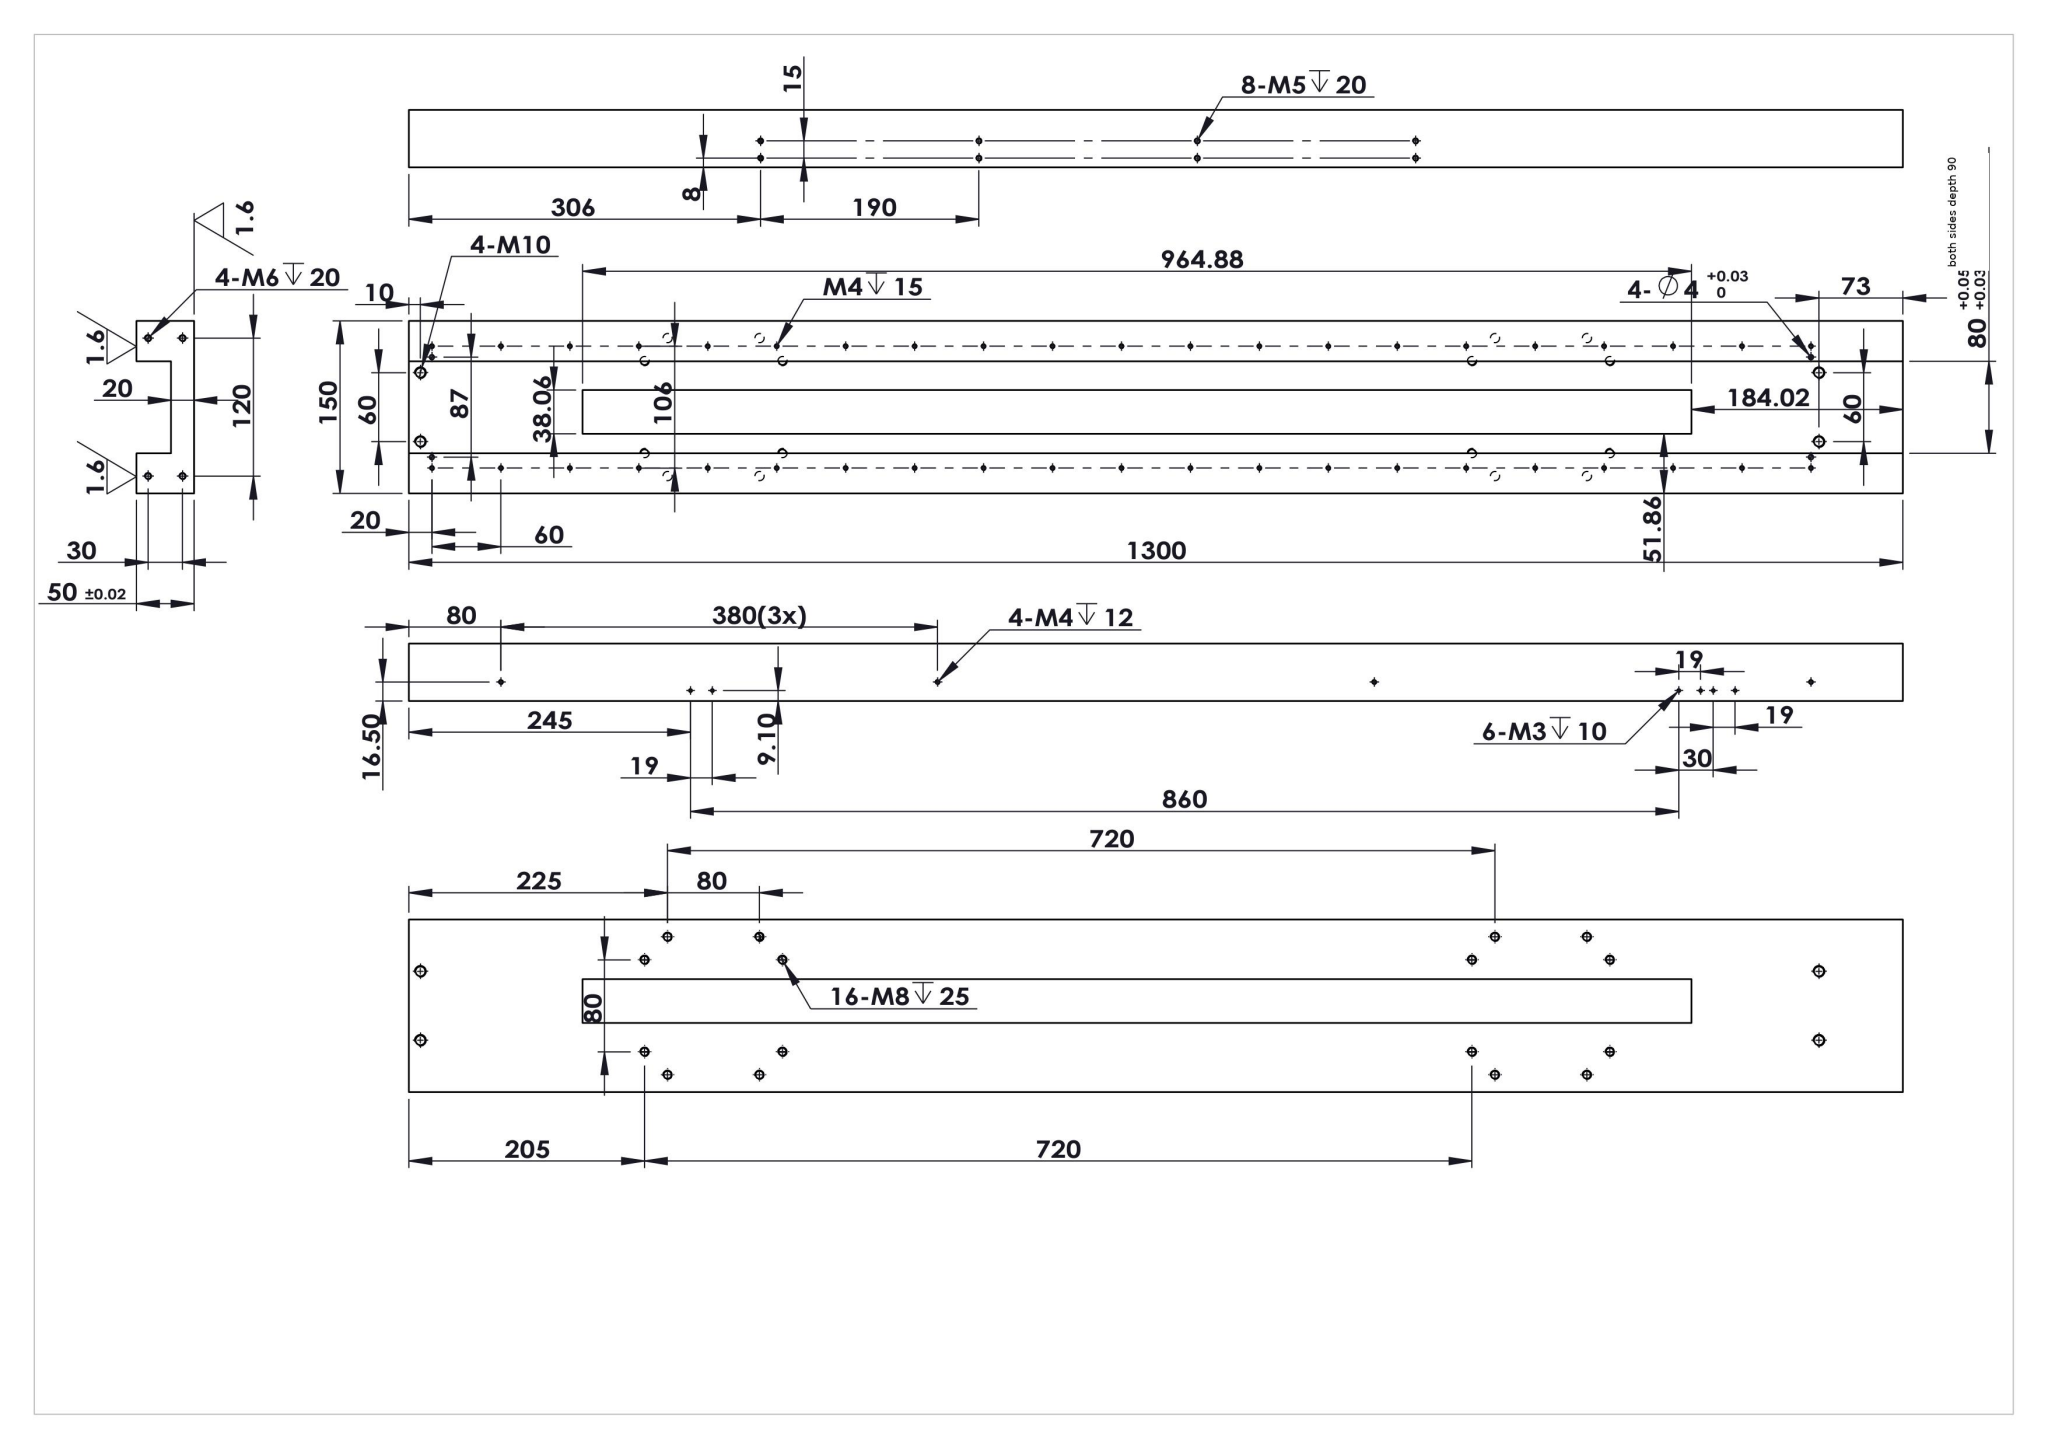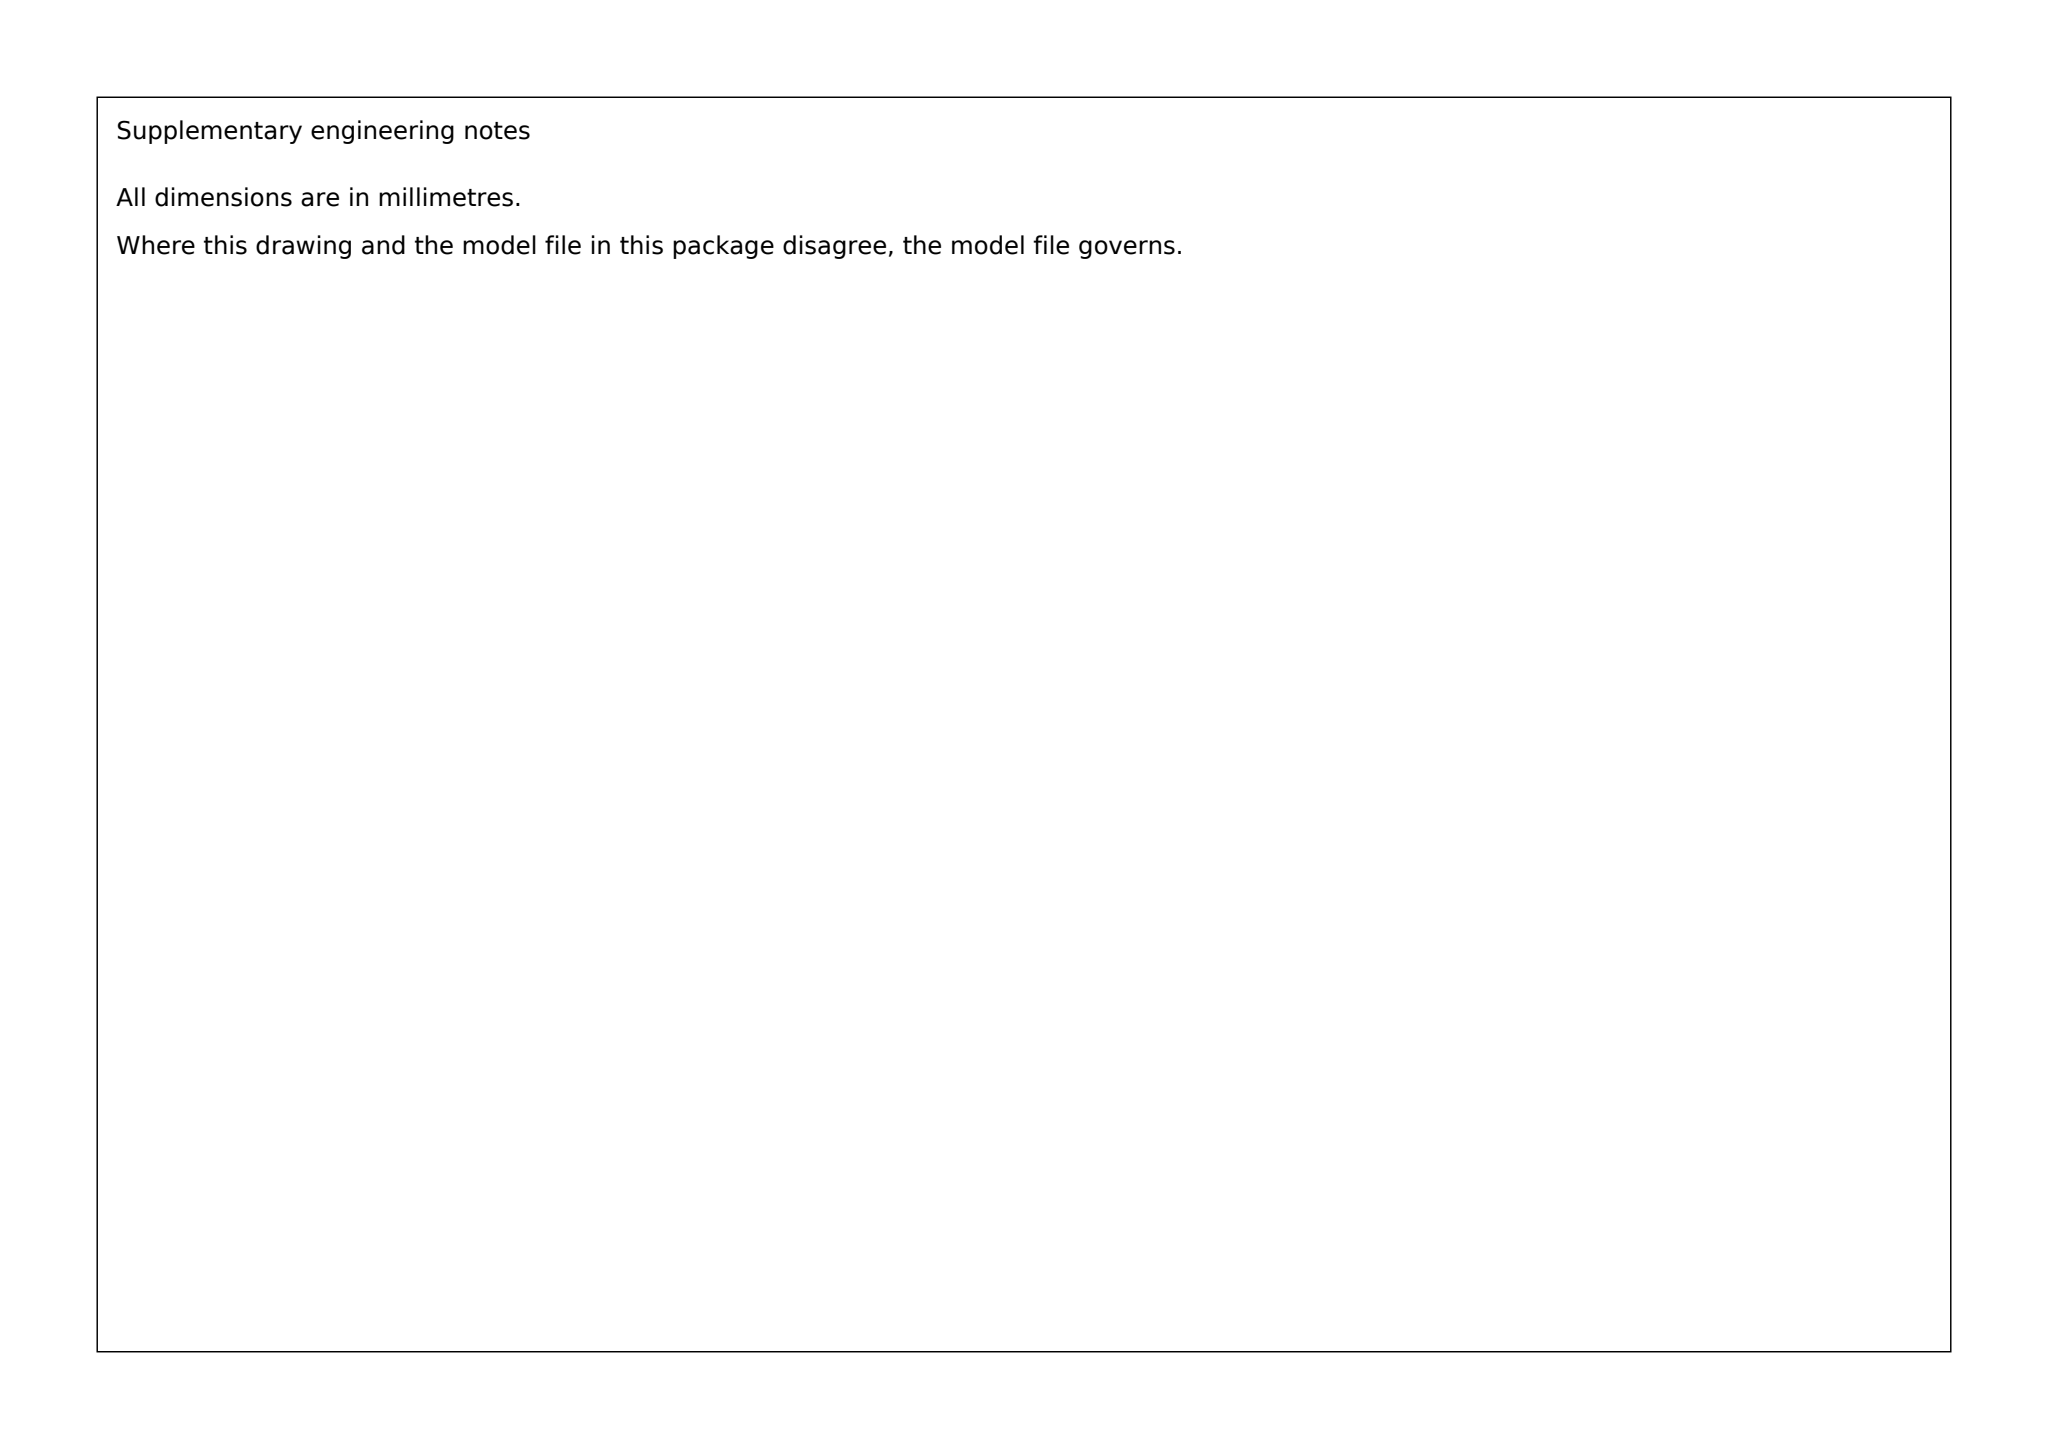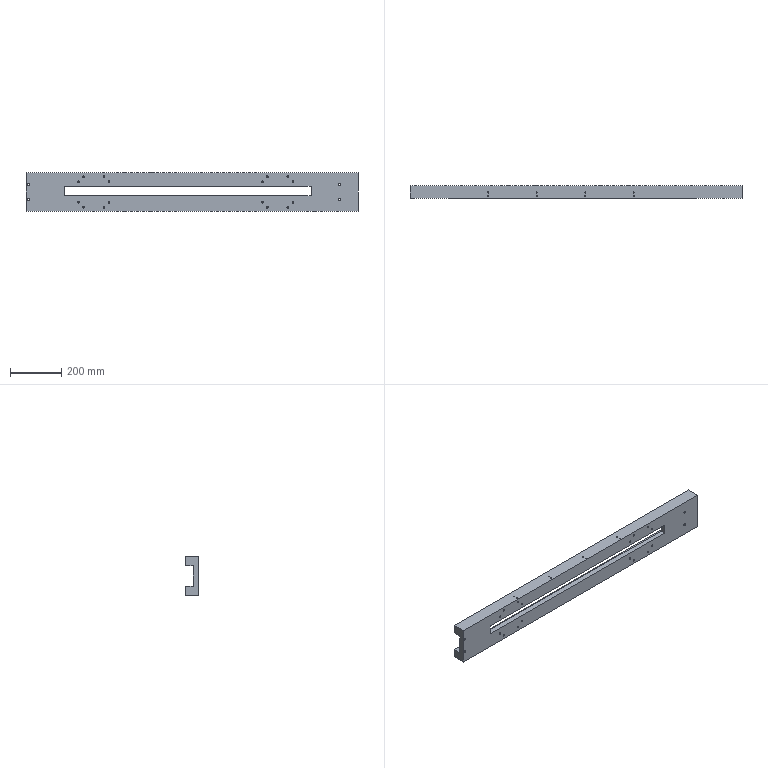Part | SolidWorks | mm | 1 solid | 355 faces | box 1300 x 50 x 150 mm | volume 5866555 mm3 | cylinder 179 | cone 158 | plane 18 | commonest cylinder face diameters 3.3 x92 6.8 x32 4.2 x19 2.5 x12 5 x8 4 x8 8.5 x8
build123d program:
from build123d import *

# Parameters (mm, degrees)
SKETCH1_2_W                = 1300
SKETCH1_2_H                = 50
BOSS_EXTRUDE1_DEPTH        = 75
SKETCH2_2_W                = 1300
SKETCH2_2_H                = 80
CUT_EXTRUDE1_2_DEPTH       = 30
M10_TAPPED_HOLE1_D         = 8.5
M4_TAPPED_HOLE1_AT_2_COUNT = 2
M4_TAPPED_HOLE1_AT_2_PITCH = 106
LPATTERN1_COUNT            = 21
LPATTERN1_PITCH            = 60
SKETCH5_R                  = 2
CUT_EXTRUDE1_DEPTH         = 10
M6_TAPPED_HOLE1_D          = 5
M6_TAPPED_HOLE1_DEPTH      = 18
M6_TAPPED_HOLE1_TIP        = 1.502
M3_TAPPED_HOLE1_D          = 2.5
M3_TAPPED_HOLE1_DEPTH      = 11.5
M3_TAPPED_HOLE1_TIP        = 0.7511
M4_TAPPED_HOLE1_2_D        = 3.3
M4_TAPPED_HOLE1_2_DEPTH    = 14.1
M4_TAPPED_HOLE1_2_TIP      = 0.9914
M5_TAPPED_HOLE1_AT_2_COUNT = 2
M5_TAPPED_HOLE1_AT_2_PITCH = 15
LPATTERN2_COUNT            = 4
LPATTERN2_PITCH            = 190
M8_TAPPED_HOLE1_D          = 6.8
M8_TAPPED_HOLE1_DEPTH      = 23.75
M8_TAPPED_HOLE1_TIP        = 2.043
SKETCH5_2_W                = 964.881
SKETCH5_2_H                = 38.06
CUT_EXTRUDE2_DEPTH         = 267


with BuildPart() as part:
    # Sketch1_2 → Boss-Extrude1 (new, symmetric)
    with BuildSketch(Plane.XY):
        Rectangle(SKETCH1_2_W, SKETCH1_2_H)
    extrude(amount=BOSS_EXTRUDE1_DEPTH, both=True)

    # Sketch2_2 → Cut-Extrude1_2 (cut)
    with BuildSketch(Plane(origin=(0, 25, 0), x_dir=(1, 0, 0), z_dir=(0, 1, 0))):
        Rectangle(SKETCH2_2_W, SKETCH2_2_H)
    extrude(amount=-CUT_EXTRUDE1_2_DEPTH, mode=Mode.SUBTRACT)

    # M10 Tapped Hole1 (through all)
    with Locations(Plane(origin=(0, -5, 0), x_dir=(1, 0, 0), z_dir=(0, 1, 0))):
        with Locations((-640, 30), (-640, -30), (577, 30), (577, -30)):
            Hole(M10_TAPPED_HOLE1_D / 2)

    # Sketch3 → M4 Tapped Hole1 (revolve, cut)
    with BuildSketch(Plane(origin=(-630, 25, -53), x_dir=(0, 0, 1), z_dir=(1, 0, 0))):
        Polygon((0, 0), (0, 18.091), (1.65, 17.1), (1.65, 0), align=None)
    m4_tapped_hole1 = revolve(axis=Axis((-630, 31.35, -53), (0, -1, 0)), mode=Mode.SUBTRACT)

    # M4 Tapped Hole1 at 2: M4 Tapped Hole1 ×2
    with Locations(*[(0, 0, i * M4_TAPPED_HOLE1_AT_2_PITCH) for i in range(1, M4_TAPPED_HOLE1_AT_2_COUNT)]):
        add(m4_tapped_hole1, mode=Mode.SUBTRACT)

    # LPattern1: M4 Tapped Hole1 ×21
    with Locations(*[(i * LPATTERN1_PITCH, 0, 0) for i in range(1, LPATTERN1_COUNT)]):
        add(m4_tapped_hole1, mode=Mode.SUBTRACT)

    # LPattern1 copy 1 sketch → LPattern1 copy 1 (revolve, cut)
    with BuildSketch(Plane(origin=(-570, 25, 53), x_dir=(0, 0, 1), z_dir=(1, 0, 0))):
        Polygon((0, 0), (0, 18.091), (1.65, 17.1), (1.65, 0), align=None)
    revolve(axis=Axis((-570, 31.35, 53), (0, -1, 0)), mode=Mode.SUBTRACT)

    # LPattern1 copy 2 sketch → LPattern1 copy 2 (revolve, cut)
    with BuildSketch(Plane(origin=(-510, 25, 53), x_dir=(0, 0, 1), z_dir=(1, 0, 0))):
        Polygon((0, 0), (0, 18.091), (1.65, 17.1), (1.65, 0), align=None)
    revolve(axis=Axis((-510, 31.35, 53), (0, -1, 0)), mode=Mode.SUBTRACT)

    # LPattern1 copy 3 sketch → LPattern1 copy 3 (revolve, cut)
    with BuildSketch(Plane(origin=(-450, 25, 53), x_dir=(0, 0, 1), z_dir=(1, 0, 0))):
        Polygon((0, 0), (0, 18.091), (1.65, 17.1), (1.65, 0), align=None)
    revolve(axis=Axis((-450, 31.35, 53), (0, -1, 0)), mode=Mode.SUBTRACT)

    # LPattern1 copy 4 sketch → LPattern1 copy 4 (revolve, cut)
    with BuildSketch(Plane(origin=(-390, 25, 53), x_dir=(0, 0, 1), z_dir=(1, 0, 0))):
        Polygon((0, 0), (0, 18.091), (1.65, 17.1), (1.65, 0), align=None)
    revolve(axis=Axis((-390, 31.35, 53), (0, -1, 0)), mode=Mode.SUBTRACT)

    # LPattern1 copy 5 sketch → LPattern1 copy 5 (revolve, cut)
    with BuildSketch(Plane(origin=(-330, 25, 53), x_dir=(0, 0, 1), z_dir=(1, 0, 0))):
        Polygon((0, 0), (0, 18.091), (1.65, 17.1), (1.65, 0), align=None)
    revolve(axis=Axis((-330, 31.35, 53), (0, -1, 0)), mode=Mode.SUBTRACT)

    # LPattern1 copy 6 sketch → LPattern1 copy 6 (revolve, cut)
    with BuildSketch(Plane(origin=(-270, 25, 53), x_dir=(0, 0, 1), z_dir=(1, 0, 0))):
        Polygon((0, 0), (0, 18.091), (1.65, 17.1), (1.65, 0), align=None)
    revolve(axis=Axis((-270, 31.35, 53), (0, -1, 0)), mode=Mode.SUBTRACT)

    # LPattern1 copy 7 sketch → LPattern1 copy 7 (revolve, cut)
    with BuildSketch(Plane(origin=(-210, 25, 53), x_dir=(0, 0, 1), z_dir=(1, 0, 0))):
        Polygon((0, 0), (0, 18.091), (1.65, 17.1), (1.65, 0), align=None)
    revolve(axis=Axis((-210, 31.35, 53), (0, -1, 0)), mode=Mode.SUBTRACT)

    # LPattern1 copy 8 sketch → LPattern1 copy 8 (revolve, cut)
    with BuildSketch(Plane(origin=(-150, 25, 53), x_dir=(0, 0, 1), z_dir=(1, 0, 0))):
        Polygon((0, 0), (0, 18.091), (1.65, 17.1), (1.65, 0), align=None)
    revolve(axis=Axis((-150, 31.35, 53), (0, -1, 0)), mode=Mode.SUBTRACT)

    # LPattern1 copy 9 sketch → LPattern1 copy 9 (revolve, cut)
    with BuildSketch(Plane(origin=(-90, 25, 53), x_dir=(0, 0, 1), z_dir=(1, 0, 0))):
        Polygon((0, 0), (0, 18.091), (1.65, 17.1), (1.65, 0), align=None)
    revolve(axis=Axis((-90, 31.35, 53), (0, -1, 0)), mode=Mode.SUBTRACT)

    # LPattern1 copy 10 sketch → LPattern1 copy 10 (revolve, cut)
    with BuildSketch(Plane(origin=(-30, 25, 53), x_dir=(0, 0, 1), z_dir=(1, 0, 0))):
        Polygon((0, 0), (0, 18.091), (1.65, 17.1), (1.65, 0), align=None)
    revolve(axis=Axis((-30, 31.35, 53), (0, -1, 0)), mode=Mode.SUBTRACT)

    # LPattern1 copy 11 sketch → LPattern1 copy 11 (revolve, cut)
    with BuildSketch(Plane(origin=(30, 25, 53), x_dir=(0, 0, 1), z_dir=(1, 0, 0))):
        Polygon((0, 0), (0, 18.091), (1.65, 17.1), (1.65, 0), align=None)
    revolve(axis=Axis((30, 31.35, 53), (0, -1, 0)), mode=Mode.SUBTRACT)

    # LPattern1 copy 12 sketch → LPattern1 copy 12 (revolve, cut)
    with BuildSketch(Plane(origin=(90, 25, 53), x_dir=(0, 0, 1), z_dir=(1, 0, 0))):
        Polygon((0, 0), (0, 18.091), (1.65, 17.1), (1.65, 0), align=None)
    revolve(axis=Axis((90, 31.35, 53), (0, -1, 0)), mode=Mode.SUBTRACT)

    # LPattern1 copy 13 sketch → LPattern1 copy 13 (revolve, cut)
    with BuildSketch(Plane(origin=(150, 25, 53), x_dir=(0, 0, 1), z_dir=(1, 0, 0))):
        Polygon((0, 0), (0, 18.091), (1.65, 17.1), (1.65, 0), align=None)
    revolve(axis=Axis((150, 31.35, 53), (0, -1, 0)), mode=Mode.SUBTRACT)

    # LPattern1 copy 14 sketch → LPattern1 copy 14 (revolve, cut)
    with BuildSketch(Plane(origin=(210, 25, 53), x_dir=(0, 0, 1), z_dir=(1, 0, 0))):
        Polygon((0, 0), (0, 18.091), (1.65, 17.1), (1.65, 0), align=None)
    revolve(axis=Axis((210, 31.35, 53), (0, -1, 0)), mode=Mode.SUBTRACT)

    # LPattern1 copy 15 sketch → LPattern1 copy 15 (revolve, cut)
    with BuildSketch(Plane(origin=(270, 25, 53), x_dir=(0, 0, 1), z_dir=(1, 0, 0))):
        Polygon((0, 0), (0, 18.091), (1.65, 17.1), (1.65, 0), align=None)
    revolve(axis=Axis((270, 31.35, 53), (0, -1, 0)), mode=Mode.SUBTRACT)

    # LPattern1 copy 16 sketch → LPattern1 copy 16 (revolve, cut)
    with BuildSketch(Plane(origin=(330, 25, 53), x_dir=(0, 0, 1), z_dir=(1, 0, 0))):
        Polygon((0, 0), (0, 18.091), (1.65, 17.1), (1.65, 0), align=None)
    revolve(axis=Axis((330, 31.35, 53), (0, -1, 0)), mode=Mode.SUBTRACT)

    # LPattern1 copy 17 sketch → LPattern1 copy 17 (revolve, cut)
    with BuildSketch(Plane(origin=(390, 25, 53), x_dir=(0, 0, 1), z_dir=(1, 0, 0))):
        Polygon((0, 0), (0, 18.091), (1.65, 17.1), (1.65, 0), align=None)
    revolve(axis=Axis((390, 31.35, 53), (0, -1, 0)), mode=Mode.SUBTRACT)

    # LPattern1 copy 18 sketch → LPattern1 copy 18 (revolve, cut)
    with BuildSketch(Plane(origin=(450, 25, 53), x_dir=(0, 0, 1), z_dir=(1, 0, 0))):
        Polygon((0, 0), (0, 18.091), (1.65, 17.1), (1.65, 0), align=None)
    revolve(axis=Axis((450, 31.35, 53), (0, -1, 0)), mode=Mode.SUBTRACT)

    # LPattern1 copy 19 sketch → LPattern1 copy 19 (revolve, cut)
    with BuildSketch(Plane(origin=(510, 25, 53), x_dir=(0, 0, 1), z_dir=(1, 0, 0))):
        Polygon((0, 0), (0, 18.091), (1.65, 17.1), (1.65, 0), align=None)
    revolve(axis=Axis((510, 31.35, 53), (0, -1, 0)), mode=Mode.SUBTRACT)

    # LPattern1 copy 20 sketch → LPattern1 copy 20 (revolve, cut)
    with BuildSketch(Plane(origin=(570, 25, 53), x_dir=(0, 0, 1), z_dir=(1, 0, 0))):
        Polygon((0, 0), (0, 18.091), (1.65, 17.1), (1.65, 0), align=None)
    revolve(axis=Axis((570, 31.35, 53), (0, -1, 0)), mode=Mode.SUBTRACT)

    # Sketch5 → Cut-Extrude1 (cut)
    with BuildSketch(Plane(origin=(0, 25, 0), x_dir=(1, 0, 0), z_dir=(0, 1, 0))):
        with Locations(Location((-630, 43.5, 0), (0, 0, 180))):
            Circle(SKETCH5_R)
        with Locations(Location((570, 43.5, 0), (0, 0, 180))):
            Circle(SKETCH5_R)
        with Locations((570, -43.5)):
            Circle(SKETCH5_R)
        with Locations((-630, -43.5)):
            Circle(SKETCH5_R)
    extrude(amount=-CUT_EXTRUDE1_DEPTH, mode=Mode.SUBTRACT)

    # M6 Tapped Hole1
    with Locations(Plane(origin=(650, 0, 0), x_dir=(0, 0, -1), z_dir=(1, 0, 0))):
        with Locations((-60, 15), (-60, -15), (60, -15), (60, 15)):
            Hole(M6_TAPPED_HOLE1_D / 2, depth=M6_TAPPED_HOLE1_DEPTH)
            with Locations((0, 0, -(M6_TAPPED_HOLE1_DEPTH + M6_TAPPED_HOLE1_TIP / 2))):  # 118° drill point
                Cone(0, M6_TAPPED_HOLE1_D / 2, M6_TAPPED_HOLE1_TIP, mode=Mode.SUBTRACT)

    # M3 Tapped Hole1
    with Locations(Plane(origin=(0, 0, -75), x_dir=(-1, 0, 0), z_dir=(0, 0, -1))):
        with Locations((-504, 15.9), (-485, 15.9), (-474, 15.9), (-455, 15.9), (386, 15.9), (405, 15.9)):
            Hole(M3_TAPPED_HOLE1_D / 2, depth=M3_TAPPED_HOLE1_DEPTH)
            with Locations((0, 0, -(M3_TAPPED_HOLE1_DEPTH + M3_TAPPED_HOLE1_TIP / 2))):  # 118° drill point
                Cone(0, M3_TAPPED_HOLE1_D / 2, M3_TAPPED_HOLE1_TIP, mode=Mode.SUBTRACT)

    # M4 Tapped Hole1_2
    with Locations(Plane(origin=(-39.67, -41.514, -75), x_dir=(1, 0, 0), z_dir=(0, 0, -1))):
        with Locations((-150.33, -50.014), (229.67, -50.014), (609.67, -50.014), (-530.33, -50.014)):
            Hole(M4_TAPPED_HOLE1_2_D / 2, depth=M4_TAPPED_HOLE1_2_DEPTH)
            with Locations((0, 0, -(M4_TAPPED_HOLE1_2_DEPTH + M4_TAPPED_HOLE1_2_TIP / 2))):  # 118° drill point
                Cone(0, M4_TAPPED_HOLE1_2_D / 2, M4_TAPPED_HOLE1_2_TIP, mode=Mode.SUBTRACT)

    # Sketch10 → M5 Tapped Hole1 (revolve, cut)
    with BuildSketch(Plane(origin=(-344, -2, 75), x_dir=(0, -1, 0), z_dir=(1, 0, 0))):
        Polygon((0, 0), (0, 18.662), (2.1, 17.4), (2.1, 0), align=None)
    m5_tapped_hole1 = revolve(axis=Axis((-344, -2, 81.35), (0, 0, -1)), mode=Mode.SUBTRACT)

    # M5 Tapped Hole1 at 2: M5 Tapped Hole1 ×2
    with Locations(*[(0, -i * M5_TAPPED_HOLE1_AT_2_PITCH, 0) for i in range(1, M5_TAPPED_HOLE1_AT_2_COUNT)]):
        add(m5_tapped_hole1, mode=Mode.SUBTRACT)

    # LPattern2: M5 Tapped Hole1 ×4
    with Locations(*[(i * LPATTERN2_PITCH, 0, 0) for i in range(1, LPATTERN2_COUNT)]):
        add(m5_tapped_hole1, mode=Mode.SUBTRACT)

    # LPattern2 copy 1 sketch → LPattern2 copy 1 (revolve, cut)
    with BuildSketch(Plane(origin=(-154, -17, 75), x_dir=(0, -1, 0), z_dir=(1, 0, 0))):
        Polygon((0, 0), (0, 18.662), (2.1, 17.4), (2.1, 0), align=None)
    revolve(axis=Axis((-154, -17, 81.35), (0, 0, -1)), mode=Mode.SUBTRACT)

    # LPattern2 copy 2 sketch → LPattern2 copy 2 (revolve, cut)
    with BuildSketch(Plane(origin=(36, -17, 75), x_dir=(0, -1, 0), z_dir=(1, 0, 0))):
        Polygon((0, 0), (0, 18.662), (2.1, 17.4), (2.1, 0), align=None)
    revolve(axis=Axis((36, -17, 81.35), (0, 0, -1)), mode=Mode.SUBTRACT)

    # LPattern2 copy 3 sketch → LPattern2 copy 3 (revolve, cut)
    with BuildSketch(Plane(origin=(226, -17, 75), x_dir=(0, -1, 0), z_dir=(1, 0, 0))):
        Polygon((0, 0), (0, 18.662), (2.1, 17.4), (2.1, 0), align=None)
    revolve(axis=Axis((226, -17, 81.35), (0, 0, -1)), mode=Mode.SUBTRACT)

    # M8 Tapped Hole1
    with Locations(Plane(origin=(0, -25, 0), x_dir=(-1, 0, 0), z_dir=(0, -1, 0))):
        with Locations((-395, -40), (-375, -60), (-295, -60), (-275, -40), (325, -40), (345, -60), (425, -60), (445, -40), (445, 40), (425, 60), (345, 60), (325, 40), (-275, 40), (-295, 60), (-375, 60), (-395, 40)):
            Hole(M8_TAPPED_HOLE1_D / 2, depth=M8_TAPPED_HOLE1_DEPTH)
            with Locations((0, 0, -(M8_TAPPED_HOLE1_DEPTH + M8_TAPPED_HOLE1_TIP / 2))):  # 118° drill point
                Cone(0, M8_TAPPED_HOLE1_D / 2, M8_TAPPED_HOLE1_TIP, mode=Mode.SUBTRACT)

    # Sketch5_2 → Cut-Extrude2 (cut)
    with BuildSketch(Plane(origin=(0, -5, 0), x_dir=(1, 0, 0), z_dir=(0, 1, 0))):
        with Locations((-16.459, -4.115)):
            Rectangle(SKETCH5_2_W, SKETCH5_2_H)
    extrude(amount=-CUT_EXTRUDE2_DEPTH, mode=Mode.SUBTRACT)


solid = part.part